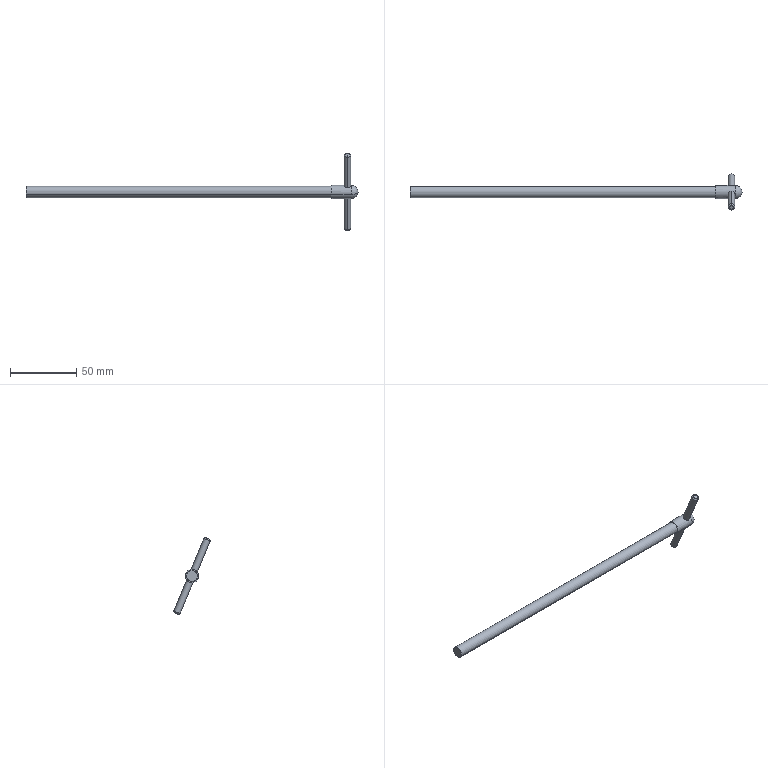Component | SolidWorks | TelescopicRod-1 | 2 solids | 20 faces | volume 15492 mm3 | cylinder 8 | torus 4 | plane 4 | cone 2 | sphere 2 | commonest cylinder face diameters 5 x4 8.5 x2 10 x2
build123d program:
from build123d import *

# Parameters (mm, degrees)
SKETCH1_R           = 5
BOSS_EXTRUDE1_DEPTH = 250
FILLET1_R           = 5
SKETCH2_R           = 2.5
CUT_EXTRUDE1_DEPTH  = 125
SKETCH3_R           = 2.5
BOSS_EXTRUDE2_DEPTH = 30.5
FILLET2_R           = 1
CHAMFER1_SIZE       = 1
SKETCH4_R           = 5.944
SKETCH4_R_2         = 4.25
CUT_EXTRUDE2_DEPTH  = 230


with BuildPart() as part:
    # Sketch1 → Boss-Extrude1 (new body)
    with BuildSketch(Plane(origin=(0, 0, 0), x_dir=(1, 0, 0), z_dir=(0, 1, 0))):
        with Locations(Location((0, 0, 0), (0, 0, 270))):
            Circle(SKETCH1_R)
    extrude(amount=BOSS_EXTRUDE1_DEPTH)

    # Fillet1
    fillet1_edges = [part.edges().sort_by_distance(p)[0] for p in [
        (0, 0, -5),
    ]]
    fillet(fillet1_edges, radius=FILLET1_R)

    # Sketch2 → Cut-Extrude1 (cut, symmetric)
    with BuildSketch(Plane(origin=(0, 0, 0), x_dir=(0, 0, -1), z_dir=(1, 0, 0))):
        with Locations((0, 8)):
            Circle(SKETCH2_R)
    extrude(amount=CUT_EXTRUDE1_DEPTH, both=True, mode=Mode.SUBTRACT)

    # Chamfer1
    chamfer1_edges = [part.edges().sort_by_distance(p)[0] for p in [
        (0, 250, -5),
    ]]
    chamfer(chamfer1_edges, length=CHAMFER1_SIZE)

    # Sketch4 → Cut-Extrude2 (cut)
    with BuildSketch(Plane(origin=(0, 250, 0), x_dir=(1, 0, 0), z_dir=(0, 1, 0))):
        Circle(SKETCH4_R)
        with Locations(Location((0, 0, 0), (0, 0, 270))):
            Circle(SKETCH4_R_2, mode=Mode.SUBTRACT)
    extrude(amount=-CUT_EXTRUDE2_DEPTH, mode=Mode.SUBTRACT)


with BuildPart() as body_2:
    # Sketch3 → Boss-Extrude2 (new, symmetric)
    with BuildSketch(Plane(origin=(0, 0, 0), x_dir=(0, 0, -1), z_dir=(1, 0, 0))):
        with Locations(Location((0, 8, 0), (0, 0, 180))):
            Circle(SKETCH3_R)
    extrude(amount=BOSS_EXTRUDE2_DEPTH, both=True)

    # Fillet2
    fillet2_edges = [body_2.edges().sort_by_distance(p)[0] for p in [
        (-30.5, 8, -2.5),
        (30.5, 8, -2.5),
    ]]
    fillet(fillet2_edges, radius=FILLET2_R)


solid = Compound([part.part, body_2.part])

# Placed as in the assembly
solid = solid.moved(Location((329.124, 2.944, 18.763), (112.448, 0, 90)))
STEP:
#1=COLOUR_RGB('',0.7922,0.8196,0.9333);
#2=FILL_AREA_STYLE_COLOUR('',#1);
#3=FILL_AREA_STYLE('',(#2));
#4=SURFACE_STYLE_FILL_AREA(#3);
#5=SURFACE_SIDE_STYLE('',(#4));
#6=SURFACE_STYLE_USAGE(.BOTH.,#5);
#7=PRESENTATION_STYLE_ASSIGNMENT((#6));
#8=CARTESIAN_POINT('',(3.115,-0.02963,0.6786));
#9=VERTEX_POINT('',#8);
#10=CARTESIAN_POINT('',(3.115,0.2615,0.7988));
#11=VERTEX_POINT('',#10);
#12=CARTESIAN_POINT('',(3.115,0.1159,0.7387));
#13=DIRECTION('',(-1.,0.,0.));
#14=DIRECTION('',(0.,-0.9242,-0.3818));
#15=AXIS2_PLACEMENT_3D('',#12,#13,#14);
#16=CIRCLE('',#15,0.1575);
#17=EDGE_CURVE('',#9,#11,#16,.T.);
#18=ORIENTED_EDGE('',*,*,#17,.F.);
#19=CARTESIAN_POINT('',(3.125,-0.03873,0.6748));
#20=VERTEX_POINT('',#19);
#21=CARTESIAN_POINT('',(3.115,-0.02963,0.6786));
#22=DIRECTION('',(0.7071,-0.6535,-0.27));
#23=VECTOR('',#22,39.37);
#24=LINE('',#21,#23);
#25=EDGE_CURVE('',#9,#20,#24,.T.);
#26=ORIENTED_EDGE('',*,*,#25,.T.);
#27=CARTESIAN_POINT('',(3.125,0.2706,0.8026));
#28=VERTEX_POINT('',#27);
#29=CARTESIAN_POINT('',(3.125,0.1159,0.7387));
#30=DIRECTION('',(-1.,0.,0.));
#31=DIRECTION('',(0.,0.9242,0.3818));
#32=AXIS2_PLACEMENT_3D('',#29,#30,#31);
#33=CIRCLE('',#32,0.1673);
#34=EDGE_CURVE('',#20,#28,#33,.T.);
#35=ORIENTED_EDGE('',*,*,#34,.T.);
#36=CARTESIAN_POINT('',(3.115,0.2615,0.7988));
#37=DIRECTION('',(0.7071,0.6535,0.27));
#38=VECTOR('',#37,39.37);
#39=LINE('',#36,#38);
#40=EDGE_CURVE('',#11,#28,#39,.T.);
#41=ORIENTED_EDGE('',*,*,#40,.F.);
#42=EDGE_LOOP('',(#18,#26,#35,#41));
#43=FACE_OUTER_BOUND('',#42,.T.);
#44=CARTESIAN_POINT('',(3.115,0.1159,0.7387));
#45=DIRECTION('',(1.,0.,0.));
#46=DIRECTION('',(0.,0.9242,0.3818));
#47=AXIS2_PLACEMENT_3D('',#44,#45,#46);
#48=CONICAL_SURFACE('',#47,0.1575,0.7854);
#49=ADVANCED_FACE('',(#43),#48,.T.);
#50=CARTESIAN_POINT('',(12.17,-0.03873,0.6748));
#51=VERTEX_POINT('',#50);
#52=CARTESIAN_POINT('',(12.17,0.2706,0.8026));
#53=VERTEX_POINT('',#52);
#54=CARTESIAN_POINT('',(12.17,0.1159,0.7387));
#55=DIRECTION('',(-1.,0.,0.));
#56=DIRECTION('',(0.,-0.9242,-0.3818));
#57=AXIS2_PLACEMENT_3D('',#54,#55,#56);
#58=CIRCLE('',#57,0.1673);
#59=EDGE_CURVE('',#51,#53,#58,.T.);
#60=ORIENTED_EDGE('',*,*,#59,.T.);
#61=CARTESIAN_POINT('',(12.17,0.2706,0.8026));
#62=DIRECTION('',(-1.,0.,0.));
#63=VECTOR('',#62,39.37);
#64=LINE('',#61,#63);
#65=EDGE_CURVE('',#53,#28,#64,.T.);
#66=ORIENTED_EDGE('',*,*,#65,.T.);
#67=ORIENTED_EDGE('',*,*,#34,.F.);
#68=CARTESIAN_POINT('',(12.17,-0.03873,0.6748));
#69=DIRECTION('',(-1.,0.,0.));
#70=VECTOR('',#69,39.37);
#71=LINE('',#68,#70);
#72=EDGE_CURVE('',#51,#20,#71,.T.);
#73=ORIENTED_EDGE('',*,*,#72,.F.);
#74=EDGE_LOOP('',(#60,#66,#67,#73));
#75=FACE_OUTER_BOUND('',#74,.T.);
#76=CARTESIAN_POINT('',(12.17,0.1159,0.7387));
#77=DIRECTION('',(-1.,0.,0.));
#78=DIRECTION('',(0.,-0.9242,-0.3818));
#79=AXIS2_PLACEMENT_3D('',#76,#77,#78);
#80=CYLINDRICAL_SURFACE('',#79,0.1673);
#81=ADVANCED_FACE('',(#75),#80,.T.);
#82=CARTESIAN_POINT('',(12.643,0.09005,0.5435));
#83=VERTEX_POINT('',#82);
#84=CARTESIAN_POINT('',(12.643,0.272,0.6187));
#85=VERTEX_POINT('',#84);
#86=CARTESIAN_POINT('',(12.643,0.09005,0.5435));
#87=CARTESIAN_POINT('',(12.649,0.09005,0.5435));
#88=CARTESIAN_POINT('',(12.656,0.09081,0.5434));
#89=CARTESIAN_POINT('',(12.669,0.09375,0.5431));
#90=CARTESIAN_POINT('',(12.675,0.09591,0.5428));
#91=CARTESIAN_POINT('',(12.687,0.1015,0.5423));
#92=CARTESIAN_POINT('',(12.692,0.1049,0.5421));
#93=CARTESIAN_POINT('',(12.703,0.1127,0.5418));
#94=CARTESIAN_POINT('',(12.708,0.1171,0.5418));
#95=CARTESIAN_POINT('',(12.717,0.1267,0.5421));
#96=CARTESIAN_POINT('',(12.721,0.1318,0.5424));
#97=CARTESIAN_POINT('',(12.728,0.1428,0.5436));
#98=CARTESIAN_POINT('',(12.731,0.1486,0.5445));
#99=CARTESIAN_POINT('',(12.736,0.1604,0.5468));
#100=CARTESIAN_POINT('',(12.738,0.1664,0.5483));
#101=CARTESIAN_POINT('',(12.74,0.1788,0.552));
#102=CARTESIAN_POINT('',(12.741,0.185,0.5542));
#103=CARTESIAN_POINT('',(12.741,0.197,0.5592));
#104=CARTESIAN_POINT('',(12.74,0.203,0.562));
#105=CARTESIAN_POINT('',(12.738,0.2144,0.5681));
#106=CARTESIAN_POINT('',(12.736,0.2197,0.5713));
#107=CARTESIAN_POINT('',(12.728,0.2349,0.5814));
#108=CARTESIAN_POINT('',(12.721,0.2436,0.5885));
#109=CARTESIAN_POINT('',(12.708,0.2541,0.5984));
#110=CARTESIAN_POINT('',(12.703,0.2571,0.6015));
#111=CARTESIAN_POINT('',(12.692,0.2624,0.6072));
#112=CARTESIAN_POINT('',(12.687,0.2647,0.6098));
#113=CARTESIAN_POINT('',(12.675,0.2683,0.614));
#114=CARTESIAN_POINT('',(12.669,0.2697,0.6157));
#115=CARTESIAN_POINT('',(12.656,0.2715,0.6181));
#116=CARTESIAN_POINT('',(12.649,0.272,0.6187));
#117=CARTESIAN_POINT('',(12.643,0.272,0.6187));
#118=B_SPLINE_CURVE_WITH_KNOTS('',3,(#86,#87,#88,#89,#90,#91,#92,#93,#94,#95,#96,#97,#98,#99,#100,#101,#102,#103,#104,#105,#106,#107,#108,#109,#110,#111,#112,#113,#114,#115,#116,#117),.UNSPECIFIED.,.F.,.F.,(4,2,2,2,2,2,2,2,2,2,2,2,2,2,2,4),(0.007951,0.008448,0.008944,0.00944,0.009936,0.01043,0.01093,0.01142,0.01192,0.01242,0.01291,0.0139,0.0144,0.0149,0.01539,0.01589),.UNSPECIFIED.);
#119=EDGE_CURVE('',#83,#85,#118,.T.);
#120=ORIENTED_EDGE('',*,*,#119,.F.);
#121=CARTESIAN_POINT('',(12.643,-0.04014,0.8587));
#122=VERTEX_POINT('',#121);
#123=CARTESIAN_POINT('',(12.643,1.904,-3.847));
#124=DIRECTION('',(0.,-0.3818,0.9242));
#125=VECTOR('',#124,39.37);
#126=LINE('',#123,#125);
#127=EDGE_CURVE('',#83,#122,#126,.T.);
#128=ORIENTED_EDGE('',*,*,#127,.T.);
#129=CARTESIAN_POINT('',(12.643,0.1418,0.9338));
#130=VERTEX_POINT('',#129);
#131=CARTESIAN_POINT('',(12.643,0.1418,0.9338));
#132=CARTESIAN_POINT('',(12.649,0.1418,0.9338));
#133=CARTESIAN_POINT('',(12.656,0.141,0.9339));
#134=CARTESIAN_POINT('',(12.669,0.1381,0.9343));
#135=CARTESIAN_POINT('',(12.675,0.1359,0.9345));
#136=CARTESIAN_POINT('',(12.693,0.1275,0.9353));
#137=CARTESIAN_POINT('',(12.703,0.1195,0.9357));
#138=CARTESIAN_POINT('',(12.717,0.1052,0.9353));
#139=CARTESIAN_POINT('',(12.721,0.09999,0.935));
#140=CARTESIAN_POINT('',(12.728,0.089,0.9338));
#141=CARTESIAN_POINT('',(12.731,0.08329,0.9329));
#142=CARTESIAN_POINT('',(12.736,0.07147,0.9305));
#143=CARTESIAN_POINT('',(12.738,0.06527,0.929));
#144=CARTESIAN_POINT('',(12.74,0.05298,0.9253));
#145=CARTESIAN_POINT('',(12.741,0.04687,0.9231));
#146=CARTESIAN_POINT('',(12.741,0.03475,0.9181));
#147=CARTESIAN_POINT('',(12.74,0.02875,0.9153));
#148=CARTESIAN_POINT('',(12.738,0.01745,0.9093));
#149=CARTESIAN_POINT('',(12.736,0.01202,0.906));
#150=CARTESIAN_POINT('',(12.731,0.001877,0.8993));
#151=CARTESIAN_POINT('',(12.728,-0.002784,0.8958));
#152=CARTESIAN_POINT('',(12.721,-0.01139,0.8889));
#153=CARTESIAN_POINT('',(12.717,-0.01533,0.8855));
#154=CARTESIAN_POINT('',(12.703,-0.02576,0.8757));
#155=CARTESIAN_POINT('',(12.692,-0.03112,0.8697));
#156=CARTESIAN_POINT('',(12.675,-0.03648,0.8633));
#157=CARTESIAN_POINT('',(12.669,-0.03786,0.8616));
#158=CARTESIAN_POINT('',(12.656,-0.03969,0.8593));
#159=CARTESIAN_POINT('',(12.649,-0.04014,0.8587));
#160=CARTESIAN_POINT('',(12.643,-0.04014,0.8587));
#161=B_SPLINE_CURVE_WITH_KNOTS('',3,(#131,#132,#133,#134,#135,#136,#137,#138,#139,#140,#141,#142,#143,#144,#145,#146,#147,#148,#149,#150,#151,#152,#153,#154,#155,#156,#157,#158,#159,#160),.UNSPECIFIED.,.F.,.F.,(4,2,2,2,2,2,2,2,2,2,2,2,2,2,4),(0.,0.000497,0.0009939,0.001988,0.002485,0.002982,0.003479,0.003976,0.004473,0.00497,0.005467,0.005964,0.006958,0.007455,0.007951),.UNSPECIFIED.);
#162=EDGE_CURVE('',#130,#122,#161,.T.);
#163=ORIENTED_EDGE('',*,*,#162,.F.);
#164=CARTESIAN_POINT('',(12.643,2.086,-3.772));
#165=DIRECTION('',(0.,-0.3818,0.9242));
#166=VECTOR('',#165,39.37);
#167=LINE('',#164,#166);
#168=EDGE_CURVE('',#85,#130,#167,.T.);
#169=ORIENTED_EDGE('',*,*,#168,.F.);
#170=EDGE_LOOP('',(#120,#128,#163,#169));
#171=FACE_OUTER_BOUND('',#170,.T.);
#172=CARTESIAN_POINT('',(12.643,1.995,-3.81));
#173=DIRECTION('',(0.,-0.3818,0.9242));
#174=DIRECTION('',(0.,0.9242,0.3818));
#175=AXIS2_PLACEMENT_3D('',#172,#173,#174);
#176=CYLINDRICAL_SURFACE('',#175,0.09843);
#177=ADVANCED_FACE('',(#171),#176,.F.);
#178=CARTESIAN_POINT('',(12.958,0.1159,0.7387));
#179=VERTEX_POINT('',#178);
#180=CARTESIAN_POINT('',(12.761,-0.06602,0.6635));
#181=VERTEX_POINT('',#180);
#182=CARTESIAN_POINT('',(12.761,0.1159,0.7387));
#183=DIRECTION('',(0.,0.3818,-0.9242));
#184=DIRECTION('',(0.,0.9242,0.3818));
#185=AXIS2_PLACEMENT_3D('',#182,#183,#184);
#186=CIRCLE('',#185,0.1969);
#187=EDGE_CURVE('',#179,#181,#186,.T.);
#188=ORIENTED_EDGE('',*,*,#187,.F.);
#189=CARTESIAN_POINT('',(12.761,0.2979,0.8139));
#190=VERTEX_POINT('',#189);
#191=CARTESIAN_POINT('',(12.761,0.1159,0.7387));
#192=DIRECTION('',(0.,-0.3818,0.9242));
#193=DIRECTION('',(0.,-0.9242,-0.3818));
#194=AXIS2_PLACEMENT_3D('',#191,#192,#193);
#195=CIRCLE('',#194,0.1969);
#196=EDGE_CURVE('',#179,#190,#195,.T.);
#197=ORIENTED_EDGE('',*,*,#196,.T.);
#198=CARTESIAN_POINT('',(12.761,0.1159,0.7387));
#199=DIRECTION('',(-1.,0.,0.));
#200=DIRECTION('',(0.,0.9242,0.3818));
#201=AXIS2_PLACEMENT_3D('',#198,#199,#200);
#202=CIRCLE('',#201,0.1969);
#203=EDGE_CURVE('',#181,#190,#202,.T.);
#204=ORIENTED_EDGE('',*,*,#203,.F.);
#205=EDGE_LOOP('',(#188,#197,#204));
#206=FACE_OUTER_BOUND('',#205,.T.);
#207=CARTESIAN_POINT('',(12.761,0.1159,0.7387));
#208=DIRECTION('',(0.,-0.3818,0.9242));
#209=DIRECTION('',(0.,-0.9242,-0.3818));
#210=AXIS2_PLACEMENT_3D('',#207,#208,#209);
#211=SPHERICAL_SURFACE('',#210,0.1969);
#212=ADVANCED_FACE('',(#206),#211,.T.);
#213=ORIENTED_EDGE('',*,*,#162,.T.);
#214=CARTESIAN_POINT('',(12.643,-0.04014,0.8587));
#215=CARTESIAN_POINT('',(12.636,-0.04014,0.8587));
#216=CARTESIAN_POINT('',(12.63,-0.03968,0.8593));
#217=CARTESIAN_POINT('',(12.617,-0.03785,0.8616));
#218=CARTESIAN_POINT('',(12.611,-0.03649,0.8633));
#219=CARTESIAN_POINT('',(12.599,-0.03286,0.8676));
#220=CARTESIAN_POINT('',(12.593,-0.03063,0.8702));
#221=CARTESIAN_POINT('',(12.583,-0.02532,0.8759));
#222=CARTESIAN_POINT('',(12.578,-0.02221,0.879));
#223=CARTESIAN_POINT('',(12.569,-0.01524,0.8856));
#224=CARTESIAN_POINT('',(12.565,-0.01137,0.8889));
#225=CARTESIAN_POINT('',(12.557,-0.002769,0.8958));
#226=CARTESIAN_POINT('',(12.554,0.001971,0.8993));
#227=CARTESIAN_POINT('',(12.549,0.012,0.906));
#228=CARTESIAN_POINT('',(12.548,0.01733,0.9092));
#229=CARTESIAN_POINT('',(12.545,0.02873,0.9153));
#230=CARTESIAN_POINT('',(12.544,0.03465,0.9181));
#231=CARTESIAN_POINT('',(12.544,0.04669,0.9231));
#232=CARTESIAN_POINT('',(12.545,0.05293,0.9253));
#233=CARTESIAN_POINT('',(12.547,0.06526,0.929));
#234=CARTESIAN_POINT('',(12.549,0.07133,0.9305));
#235=CARTESIAN_POINT('',(12.557,0.08922,0.9341));
#236=CARTESIAN_POINT('',(12.564,0.1004,0.9352));
#237=CARTESIAN_POINT('',(12.578,0.1148,0.9356));
#238=CARTESIAN_POINT('',(12.583,0.1191,0.9356));
#239=CARTESIAN_POINT('',(12.593,0.1269,0.9353));
#240=CARTESIAN_POINT('',(12.599,0.1303,0.935));
#241=CARTESIAN_POINT('',(12.611,0.1359,0.9345));
#242=CARTESIAN_POINT('',(12.617,0.1381,0.9343));
#243=CARTESIAN_POINT('',(12.629,0.141,0.9339));
#244=CARTESIAN_POINT('',(12.636,0.1418,0.9338));
#245=CARTESIAN_POINT('',(12.643,0.1418,0.9338));
#246=B_SPLINE_CURVE_WITH_KNOTS('',3,(#214,#215,#216,#217,#218,#219,#220,#221,#222,#223,#224,#225,#226,#227,#228,#229,#230,#231,#232,#233,#234,#235,#236,#237,#238,#239,#240,#241,#242,#243,#244,#245),.UNSPECIFIED.,.F.,.F.,(4,2,2,2,2,2,2,2,2,2,2,2,2,2,2,4),(0.007951,0.008448,0.008944,0.00944,0.009936,0.01043,0.01093,0.01142,0.01192,0.01242,0.01291,0.0139,0.0144,0.0149,0.01539,0.01589),.UNSPECIFIED.);
#247=EDGE_CURVE('',#122,#130,#246,.T.);
#248=ORIENTED_EDGE('',*,*,#247,.T.);
#249=EDGE_LOOP('',(#213,#248));
#250=FACE_BOUND('',#249,.T.);
#251=CARTESIAN_POINT('',(12.17,-0.06602,0.6635));
#252=VERTEX_POINT('',#251);
#253=CARTESIAN_POINT('',(12.17,0.2979,0.8139));
#254=VERTEX_POINT('',#253);
#255=CARTESIAN_POINT('',(12.17,0.1159,0.7387));
#256=DIRECTION('',(-1.,0.,0.));
#257=DIRECTION('',(0.,-0.9242,-0.3818));
#258=AXIS2_PLACEMENT_3D('',#255,#256,#257);
#259=CIRCLE('',#258,0.1969);
#260=EDGE_CURVE('',#252,#254,#259,.T.);
#261=ORIENTED_EDGE('',*,*,#260,.F.);
#262=CARTESIAN_POINT('',(3.115,-0.06602,0.6635));
#263=DIRECTION('',(1.,0.,0.));
#264=VECTOR('',#263,39.37);
#265=LINE('',#262,#264);
#266=EDGE_CURVE('',#252,#181,#265,.T.);
#267=ORIENTED_EDGE('',*,*,#266,.T.);
#268=ORIENTED_EDGE('',*,*,#203,.T.);
#269=CARTESIAN_POINT('',(3.115,0.2979,0.8139));
#270=DIRECTION('',(1.,0.,0.));
#271=VECTOR('',#270,39.37);
#272=LINE('',#269,#271);
#273=EDGE_CURVE('',#254,#190,#272,.T.);
#274=ORIENTED_EDGE('',*,*,#273,.F.);
#275=EDGE_LOOP('',(#261,#267,#268,#274));
#276=FACE_OUTER_BOUND('',#275,.T.);
#277=CARTESIAN_POINT('',(3.115,0.1159,0.7387));
#278=DIRECTION('',(1.,0.,0.));
#279=DIRECTION('',(0.,0.9242,0.3818));
#280=AXIS2_PLACEMENT_3D('',#277,#278,#279);
#281=CYLINDRICAL_SURFACE('',#280,0.1969);
#282=ADVANCED_FACE('',(#250,#276),#281,.T.);
#283=ORIENTED_EDGE('',*,*,#266,.F.);
#284=CARTESIAN_POINT('',(12.17,0.1159,0.7387));
#285=DIRECTION('',(-1.,0.,0.));
#286=DIRECTION('',(0.,-0.9242,-0.3818));
#287=AXIS2_PLACEMENT_3D('',#284,#285,#286);
#288=CIRCLE('',#287,0.1969);
#289=EDGE_CURVE('',#254,#252,#288,.T.);
#290=ORIENTED_EDGE('',*,*,#289,.F.);
#291=ORIENTED_EDGE('',*,*,#273,.T.);
#292=CARTESIAN_POINT('',(12.761,0.1159,0.7387));
#293=DIRECTION('',(-1.,0.,0.));
#294=DIRECTION('',(0.,0.9242,0.3818));
#295=AXIS2_PLACEMENT_3D('',#292,#293,#294);
#296=CIRCLE('',#295,0.1969);
#297=EDGE_CURVE('',#190,#181,#296,.T.);
#298=ORIENTED_EDGE('',*,*,#297,.T.);
#299=EDGE_LOOP('',(#283,#290,#291,#298));
#300=FACE_OUTER_BOUND('',#299,.T.);
#301=CARTESIAN_POINT('',(12.643,0.272,0.6187));
#302=CARTESIAN_POINT('',(12.636,0.272,0.6187));
#303=CARTESIAN_POINT('',(12.63,0.2715,0.6181));
#304=CARTESIAN_POINT('',(12.617,0.2697,0.6158));
#305=CARTESIAN_POINT('',(12.611,0.2683,0.6141));
#306=CARTESIAN_POINT('',(12.593,0.2629,0.6076));
#307=CARTESIAN_POINT('',(12.582,0.2575,0.6016));
#308=CARTESIAN_POINT('',(12.569,0.2471,0.5918));
#309=CARTESIAN_POINT('',(12.565,0.2432,0.5884));
#310=CARTESIAN_POINT('',(12.557,0.2345,0.5815));
#311=CARTESIAN_POINT('',(12.554,0.2299,0.5781));
#312=CARTESIAN_POINT('',(12.549,0.2199,0.5714));
#313=CARTESIAN_POINT('',(12.547,0.2144,0.5681));
#314=CARTESIAN_POINT('',(12.545,0.2031,0.5621));
#315=CARTESIAN_POINT('',(12.544,0.1972,0.5593));
#316=CARTESIAN_POINT('',(12.544,0.1851,0.5543));
#317=CARTESIAN_POINT('',(12.545,0.1788,0.5521));
#318=CARTESIAN_POINT('',(12.547,0.1666,0.5484));
#319=CARTESIAN_POINT('',(12.549,0.1604,0.5468));
#320=CARTESIAN_POINT('',(12.554,0.1485,0.5445));
#321=CARTESIAN_POINT('',(12.557,0.1427,0.5436));
#322=CARTESIAN_POINT('',(12.565,0.1318,0.5424));
#323=CARTESIAN_POINT('',(12.569,0.1266,0.5421));
#324=CARTESIAN_POINT('',(12.582,0.1123,0.5416));
#325=CARTESIAN_POINT('',(12.593,0.1042,0.5421));
#326=CARTESIAN_POINT('',(12.611,0.09592,0.5428));
#327=CARTESIAN_POINT('',(12.617,0.09373,0.5431));
#328=CARTESIAN_POINT('',(12.63,0.09079,0.5434));
#329=CARTESIAN_POINT('',(12.636,0.09005,0.5435));
#330=CARTESIAN_POINT('',(12.643,0.09005,0.5435));
#331=B_SPLINE_CURVE_WITH_KNOTS('',3,(#301,#302,#303,#304,#305,#306,#307,#308,#309,#310,#311,#312,#313,#314,#315,#316,#317,#318,#319,#320,#321,#322,#323,#324,#325,#326,#327,#328,#329,#330),.UNSPECIFIED.,.F.,.F.,(4,2,2,2,2,2,2,2,2,2,2,2,2,2,4),(0.,0.000497,0.0009939,0.001988,0.002485,0.002982,0.003479,0.003976,0.004473,0.00497,0.005467,0.005964,0.006958,0.007455,0.007951),.UNSPECIFIED.);
#332=EDGE_CURVE('',#85,#83,#331,.T.);
#333=ORIENTED_EDGE('',*,*,#332,.T.);
#334=ORIENTED_EDGE('',*,*,#119,.T.);
#335=EDGE_LOOP('',(#333,#334));
#336=FACE_BOUND('',#335,.T.);
#337=CARTESIAN_POINT('',(3.115,0.1159,0.7387));
#338=DIRECTION('',(1.,0.,0.));
#339=DIRECTION('',(0.,0.9242,0.3818));
#340=AXIS2_PLACEMENT_3D('',#337,#338,#339);
#341=CYLINDRICAL_SURFACE('',#340,0.1969);
#342=ADVANCED_FACE('',(#300,#336),#341,.T.);
#343=ORIENTED_EDGE('',*,*,#196,.F.);
#344=ORIENTED_EDGE('',*,*,#187,.T.);
#345=ORIENTED_EDGE('',*,*,#297,.F.);
#346=EDGE_LOOP('',(#343,#344,#345));
#347=FACE_OUTER_BOUND('',#346,.T.);
#348=CARTESIAN_POINT('',(12.761,0.1159,0.7387));
#349=DIRECTION('',(0.,-0.3818,0.9242));
#350=DIRECTION('',(0.,-0.9242,-0.3818));
#351=AXIS2_PLACEMENT_3D('',#348,#349,#350);
#352=SPHERICAL_SURFACE('',#351,0.1969);
#353=ADVANCED_FACE('',(#347),#352,.T.);
#354=ORIENTED_EDGE('',*,*,#127,.F.);
#355=ORIENTED_EDGE('',*,*,#332,.F.);
#356=ORIENTED_EDGE('',*,*,#168,.T.);
#357=ORIENTED_EDGE('',*,*,#247,.F.);
#358=EDGE_LOOP('',(#354,#355,#356,#357));
#359=FACE_OUTER_BOUND('',#358,.T.);
#360=CARTESIAN_POINT('',(12.643,1.995,-3.81));
#361=DIRECTION('',(0.,-0.3818,0.9242));
#362=DIRECTION('',(0.,0.9242,0.3818));
#363=AXIS2_PLACEMENT_3D('',#360,#361,#362);
#364=CYLINDRICAL_SURFACE('',#363,0.09843);
#365=ADVANCED_FACE('',(#359),#364,.F.);
#366=ORIENTED_EDGE('',*,*,#59,.F.);
#367=CARTESIAN_POINT('',(12.17,0.1159,0.7387));
#368=DIRECTION('',(-1.,0.,0.));
#369=DIRECTION('',(0.,-0.9242,-0.3818));
#370=AXIS2_PLACEMENT_3D('',#367,#368,#369);
#371=CIRCLE('',#370,0.1673);
#372=EDGE_CURVE('',#53,#51,#371,.T.);
#373=ORIENTED_EDGE('',*,*,#372,.F.);
#374=EDGE_LOOP('',(#366,#373));
#375=FACE_BOUND('',#374,.T.);
#376=ORIENTED_EDGE('',*,*,#289,.T.);
#377=ORIENTED_EDGE('',*,*,#260,.T.);
#378=EDGE_LOOP('',(#376,#377));
#379=FACE_OUTER_BOUND('',#378,.T.);
#380=CARTESIAN_POINT('',(12.17,0.1159,0.7387));
#381=DIRECTION('',(-1.,0.,0.));
#382=DIRECTION('',(0.,-0.9242,-0.3818));
#383=AXIS2_PLACEMENT_3D('',#380,#381,#382);
#384=PLANE('',#383);
#385=ADVANCED_FACE('',(#375,#379),#384,.T.);
#386=ORIENTED_EDGE('',*,*,#65,.F.);
#387=ORIENTED_EDGE('',*,*,#372,.T.);
#388=ORIENTED_EDGE('',*,*,#72,.T.);
#389=CARTESIAN_POINT('',(3.125,0.1159,0.7387));
#390=DIRECTION('',(-1.,0.,0.));
#391=DIRECTION('',(0.,0.9242,0.3818));
#392=AXIS2_PLACEMENT_3D('',#389,#390,#391);
#393=CIRCLE('',#392,0.1673);
#394=EDGE_CURVE('',#28,#20,#393,.T.);
#395=ORIENTED_EDGE('',*,*,#394,.F.);
#396=EDGE_LOOP('',(#386,#387,#388,#395));
#397=FACE_OUTER_BOUND('',#396,.T.);
#398=CARTESIAN_POINT('',(12.17,0.1159,0.7387));
#399=DIRECTION('',(-1.,0.,0.));
#400=DIRECTION('',(0.,-0.9242,-0.3818));
#401=AXIS2_PLACEMENT_3D('',#398,#399,#400);
#402=CYLINDRICAL_SURFACE('',#401,0.1673);
#403=ADVANCED_FACE('',(#397),#402,.T.);
#404=CARTESIAN_POINT('',(3.115,0.1159,0.7387));
#405=DIRECTION('',(-1.,0.,0.));
#406=DIRECTION('',(0.,-0.9242,-0.3818));
#407=AXIS2_PLACEMENT_3D('',#404,#405,#406);
#408=CIRCLE('',#407,0.1575);
#409=EDGE_CURVE('',#11,#9,#408,.T.);
#410=ORIENTED_EDGE('',*,*,#409,.T.);
#411=ORIENTED_EDGE('',*,*,#17,.T.);
#412=EDGE_LOOP('',(#410,#411));
#413=FACE_OUTER_BOUND('',#412,.T.);
#414=CARTESIAN_POINT('',(3.115,0.1159,0.7387));
#415=DIRECTION('',(-1.,0.,0.));
#416=DIRECTION('',(0.,-0.9242,-0.3818));
#417=AXIS2_PLACEMENT_3D('',#414,#415,#416);
#418=PLANE('',#417);
#419=ADVANCED_FACE('',(#413),#418,.T.);
#420=ORIENTED_EDGE('',*,*,#25,.F.);
#421=ORIENTED_EDGE('',*,*,#409,.F.);
#422=ORIENTED_EDGE('',*,*,#40,.T.);
#423=ORIENTED_EDGE('',*,*,#394,.T.);
#424=EDGE_LOOP('',(#420,#421,#422,#423));
#425=FACE_OUTER_BOUND('',#424,.T.);
#426=CARTESIAN_POINT('',(3.115,0.1159,0.7387));
#427=DIRECTION('',(1.,0.,0.));
#428=DIRECTION('',(0.,0.9242,0.3818));
#429=AXIS2_PLACEMENT_3D('',#426,#427,#428);
#430=CONICAL_SURFACE('',#429,0.1575,0.7854);
#431=ADVANCED_FACE('',(#425),#430,.T.);
#432=CLOSED_SHELL('',(#49,#81,#177,#212,#282,#342,#353,#365,#385,#403,#419,#431));
#433=MANIFOLD_SOLID_BREP('',#432);
#434=STYLED_ITEM('',(#7),#433);
#435=(LENGTH_UNIT()NAMED_UNIT(*)SI_UNIT($,.METRE.));
#436=LENGTH_MEASURE_WITH_UNIT(LENGTH_MEASURE(0.0254),#435);
#437=DIMENSIONAL_EXPONENTS(1.,0.,0.,0.,0.,0.,0.);
#438=(CONVERSION_BASED_UNIT('',#436)LENGTH_UNIT()NAMED_UNIT(#437));
#439=UNCERTAINTY_MEASURE_WITH_UNIT(LENGTH_MEASURE(0.00001),#438,'','');
#440=(NAMED_UNIT(*)PLANE_ANGLE_UNIT()SI_UNIT($,.RADIAN.));
#441=(NAMED_UNIT(*)SI_UNIT($,.STERADIAN.)SOLID_ANGLE_UNIT());
#442=(GEOMETRIC_REPRESENTATION_CONTEXT(3)GLOBAL_UNCERTAINTY_ASSIGNED_CONTEXT((#439))GLOBAL_UNIT_ASSIGNED_CONTEXT((#438,#440,#441))REPRESENTATION_CONTEXT('',''));
#443=MECHANICAL_DESIGN_GEOMETRIC_PRESENTATION_REPRESENTATION('',(#434),#442);
#444=PRESENTATION_LAYER_ASSIGNMENT('','',(#434));
#445=COLOUR_RGB('',0.7922,0.8196,0.9333);
#446=FILL_AREA_STYLE_COLOUR('',#445);
#447=FILL_AREA_STYLE('',(#446));
#448=SURFACE_STYLE_FILL_AREA(#447);
#449=SURFACE_SIDE_STYLE('',(#448));
#450=SURFACE_STYLE_USAGE(.BOTH.,#449);
#451=PRESENTATION_STYLE_ASSIGNMENT((#450));
#452=CARTESIAN_POINT('',(12.643,-0.4185,1.775));
#453=VERTEX_POINT('',#452);
#454=CARTESIAN_POINT('',(12.643,-0.2366,1.85));
#455=VERTEX_POINT('',#454);
#456=CARTESIAN_POINT('',(12.643,-0.3276,1.812));
#457=DIRECTION('',(0.,0.3818,-0.9242));
#458=DIRECTION('',(0.,0.9242,0.3818));
#459=AXIS2_PLACEMENT_3D('',#456,#457,#458);
#460=CIRCLE('',#459,0.09843);
#461=EDGE_CURVE('',#453,#455,#460,.T.);
#462=ORIENTED_EDGE('',*,*,#461,.F.);
#463=CARTESIAN_POINT('',(12.643,-0.3972,1.826));
#464=VERTEX_POINT('',#463);
#465=CARTESIAN_POINT('',(12.643,-0.3821,1.79));
#466=DIRECTION('',(-1.,0.,0.));
#467=DIRECTION('',(0.,-1.,0.));
#468=AXIS2_PLACEMENT_3D('',#465,#466,#467);
#469=CIRCLE('',#468,0.03937);
#470=EDGE_CURVE('',#453,#464,#469,.T.);
#471=ORIENTED_EDGE('',*,*,#470,.T.);
#472=CARTESIAN_POINT('',(12.643,-0.288,1.871));
#473=VERTEX_POINT('',#472);
#474=CARTESIAN_POINT('',(12.643,-0.3426,1.848));
#475=DIRECTION('',(0.,-0.3818,0.9242));
#476=DIRECTION('',(0.,0.9242,0.3818));
#477=AXIS2_PLACEMENT_3D('',#474,#475,#476);
#478=CIRCLE('',#477,0.05906);
#479=EDGE_CURVE('',#473,#464,#478,.T.);
#480=ORIENTED_EDGE('',*,*,#479,.F.);
#481=CARTESIAN_POINT('',(12.643,-0.273,1.835));
#482=DIRECTION('',(1.,0.,0.));
#483=DIRECTION('',(0.,0.,-1.));
#484=AXIS2_PLACEMENT_3D('',#481,#482,#483);
#485=CIRCLE('',#484,0.03937);
#486=EDGE_CURVE('',#455,#473,#485,.T.);
#487=ORIENTED_EDGE('',*,*,#486,.F.);
#488=EDGE_LOOP('',(#462,#471,#480,#487));
#489=FACE_OUTER_BOUND('',#488,.T.);
#490=CARTESIAN_POINT('',(12.643,-0.3276,1.812));
#491=DIRECTION('',(0.,-0.3818,0.9242));
#492=DIRECTION('',(0.,0.9242,0.3818));
#493=AXIS2_PLACEMENT_3D('',#490,#491,#492);
#494=TOROIDAL_SURFACE('',#493,0.05906,0.03937);
#495=ADVANCED_FACE('',(#489),#494,.T.);
#496=CARTESIAN_POINT('',(12.643,0.5199,-0.3937));
#497=VERTEX_POINT('',#496);
#498=CARTESIAN_POINT('',(12.643,0.629,-0.3486));
#499=VERTEX_POINT('',#498);
#500=CARTESIAN_POINT('',(12.643,0.5744,-0.3711));
#501=DIRECTION('',(0.,0.3818,-0.9242));
#502=DIRECTION('',(0.,0.9242,0.3818));
#503=AXIS2_PLACEMENT_3D('',#500,#501,#502);
#504=CIRCLE('',#503,0.05906);
#505=EDGE_CURVE('',#497,#499,#504,.T.);
#506=ORIENTED_EDGE('',*,*,#505,.F.);
#507=CARTESIAN_POINT('',(12.643,0.4684,-0.3723));
#508=VERTEX_POINT('',#507);
#509=CARTESIAN_POINT('',(12.643,0.5048,-0.3573));
#510=DIRECTION('',(-1.,0.,0.));
#511=DIRECTION('',(0.,-1.,0.));
#512=AXIS2_PLACEMENT_3D('',#509,#510,#511);
#513=CIRCLE('',#512,0.03937);
#514=EDGE_CURVE('',#497,#508,#513,.T.);
#515=ORIENTED_EDGE('',*,*,#514,.T.);
#516=CARTESIAN_POINT('',(12.643,0.6504,-0.2971));
#517=VERTEX_POINT('',#516);
#518=CARTESIAN_POINT('',(12.643,0.5594,-0.3347));
#519=DIRECTION('',(0.,-0.3818,0.9242));
#520=DIRECTION('',(0.,0.9242,0.3818));
#521=AXIS2_PLACEMENT_3D('',#518,#519,#520);
#522=CIRCLE('',#521,0.09843);
#523=EDGE_CURVE('',#517,#508,#522,.T.);
#524=ORIENTED_EDGE('',*,*,#523,.F.);
#525=CARTESIAN_POINT('',(12.643,0.614,-0.3122));
#526=DIRECTION('',(1.,0.,0.));
#527=DIRECTION('',(0.,0.,-1.));
#528=AXIS2_PLACEMENT_3D('',#525,#526,#527);
#529=CIRCLE('',#528,0.03937);
#530=EDGE_CURVE('',#499,#517,#529,.T.);
#531=ORIENTED_EDGE('',*,*,#530,.F.);
#532=EDGE_LOOP('',(#506,#515,#524,#531));
#533=FACE_OUTER_BOUND('',#532,.T.);
#534=CARTESIAN_POINT('',(12.643,0.5594,-0.3347));
#535=DIRECTION('',(0.,-0.3818,0.9242));
#536=DIRECTION('',(0.,0.9242,0.3818));
#537=AXIS2_PLACEMENT_3D('',#534,#535,#536);
#538=TOROIDAL_SURFACE('',#537,0.05906,0.03937);
#539=ADVANCED_FACE('',(#533),#538,.T.);
#540=ORIENTED_EDGE('',*,*,#461,.T.);
#541=CARTESIAN_POINT('',(12.643,-0.2516,1.886));
#542=DIRECTION('',(0.,0.3818,-0.9242));
#543=VECTOR('',#542,39.37);
#544=LINE('',#541,#543);
#545=EDGE_CURVE('',#455,#517,#544,.T.);
#546=ORIENTED_EDGE('',*,*,#545,.T.);
#547=ORIENTED_EDGE('',*,*,#523,.T.);
#548=CARTESIAN_POINT('',(12.643,-0.4336,1.811));
#549=DIRECTION('',(0.,0.3818,-0.9242));
#550=VECTOR('',#549,39.37);
#551=LINE('',#548,#550);
#552=EDGE_CURVE('',#453,#508,#551,.T.);
#553=ORIENTED_EDGE('',*,*,#552,.F.);
#554=EDGE_LOOP('',(#540,#546,#547,#553));
#555=FACE_OUTER_BOUND('',#554,.T.);
#556=CARTESIAN_POINT('',(12.643,-0.3426,1.848));
#557=DIRECTION('',(0.,0.3818,-0.9242));
#558=DIRECTION('',(0.,-0.9242,-0.3818));
#559=AXIS2_PLACEMENT_3D('',#556,#557,#558);
#560=CYLINDRICAL_SURFACE('',#559,0.09843);
#561=ADVANCED_FACE('',(#555),#560,.T.);
#562=ORIENTED_EDGE('',*,*,#545,.F.);
#563=CARTESIAN_POINT('',(12.643,-0.3276,1.812));
#564=DIRECTION('',(0.,0.3818,-0.9242));
#565=DIRECTION('',(0.,0.9242,0.3818));
#566=AXIS2_PLACEMENT_3D('',#563,#564,#565);
#567=CIRCLE('',#566,0.09843);
#568=EDGE_CURVE('',#455,#453,#567,.T.);
#569=ORIENTED_EDGE('',*,*,#568,.T.);
#570=ORIENTED_EDGE('',*,*,#552,.T.);
#571=CARTESIAN_POINT('',(12.643,0.5594,-0.3347));
#572=DIRECTION('',(0.,-0.3818,0.9242));
#573=DIRECTION('',(0.,0.9242,0.3818));
#574=AXIS2_PLACEMENT_3D('',#571,#572,#573);
#575=CIRCLE('',#574,0.09843);
#576=EDGE_CURVE('',#508,#517,#575,.T.);
#577=ORIENTED_EDGE('',*,*,#576,.T.);
#578=EDGE_LOOP('',(#562,#569,#570,#577));
#579=FACE_OUTER_BOUND('',#578,.T.);
#580=CARTESIAN_POINT('',(12.643,-0.3426,1.848));
#581=DIRECTION('',(0.,0.3818,-0.9242));
#582=DIRECTION('',(0.,-0.9242,-0.3818));
#583=AXIS2_PLACEMENT_3D('',#580,#581,#582);
#584=CYLINDRICAL_SURFACE('',#583,0.09843);
#585=ADVANCED_FACE('',(#579),#584,.T.);
#586=ORIENTED_EDGE('',*,*,#479,.T.);
#587=CARTESIAN_POINT('',(12.643,-0.3426,1.848));
#588=DIRECTION('',(0.,-0.3818,0.9242));
#589=DIRECTION('',(0.,0.9242,0.3818));
#590=AXIS2_PLACEMENT_3D('',#587,#588,#589);
#591=CIRCLE('',#590,0.05906);
#592=EDGE_CURVE('',#464,#473,#591,.T.);
#593=ORIENTED_EDGE('',*,*,#592,.T.);
#594=EDGE_LOOP('',(#586,#593));
#595=FACE_OUTER_BOUND('',#594,.T.);
#596=CARTESIAN_POINT('',(12.643,-0.3426,1.848));
#597=DIRECTION('',(0.,-0.3818,0.9242));
#598=DIRECTION('',(0.,0.9242,0.3818));
#599=AXIS2_PLACEMENT_3D('',#596,#597,#598);
#600=PLANE('',#599);
#601=ADVANCED_FACE('',(#595),#600,.T.);
#602=CARTESIAN_POINT('',(12.643,0.5744,-0.3711));
#603=DIRECTION('',(0.,0.3818,-0.9242));
#604=DIRECTION('',(0.,0.9242,0.3818));
#605=AXIS2_PLACEMENT_3D('',#602,#603,#604);
#606=CIRCLE('',#605,0.05906);
#607=EDGE_CURVE('',#499,#497,#606,.T.);
#608=ORIENTED_EDGE('',*,*,#607,.T.);
#609=ORIENTED_EDGE('',*,*,#505,.T.);
#610=EDGE_LOOP('',(#608,#609));
#611=FACE_OUTER_BOUND('',#610,.T.);
#612=CARTESIAN_POINT('',(12.643,0.5744,-0.3711));
#613=DIRECTION('',(0.,-0.3818,0.9242));
#614=DIRECTION('',(0.,0.9242,0.3818));
#615=AXIS2_PLACEMENT_3D('',#612,#613,#614);
#616=PLANE('',#615);
#617=ADVANCED_FACE('',(#611),#616,.F.);
#618=ORIENTED_EDGE('',*,*,#514,.F.);
#619=ORIENTED_EDGE('',*,*,#607,.F.);
#620=ORIENTED_EDGE('',*,*,#530,.T.);
#621=ORIENTED_EDGE('',*,*,#576,.F.);
#622=EDGE_LOOP('',(#618,#619,#620,#621));
#623=FACE_OUTER_BOUND('',#622,.T.);
#624=CARTESIAN_POINT('',(12.643,0.5594,-0.3347));
#625=DIRECTION('',(0.,-0.3818,0.9242));
#626=DIRECTION('',(0.,0.9242,0.3818));
#627=AXIS2_PLACEMENT_3D('',#624,#625,#626);
#628=TOROIDAL_SURFACE('',#627,0.05906,0.03937);
#629=ADVANCED_FACE('',(#623),#628,.T.);
#630=ORIENTED_EDGE('',*,*,#470,.F.);
#631=ORIENTED_EDGE('',*,*,#568,.F.);
#632=ORIENTED_EDGE('',*,*,#486,.T.);
#633=ORIENTED_EDGE('',*,*,#592,.F.);
#634=EDGE_LOOP('',(#630,#631,#632,#633));
#635=FACE_OUTER_BOUND('',#634,.T.);
#636=CARTESIAN_POINT('',(12.643,-0.3276,1.812));
#637=DIRECTION('',(0.,-0.3818,0.9242));
#638=DIRECTION('',(0.,0.9242,0.3818));
#639=AXIS2_PLACEMENT_3D('',#636,#637,#638);
#640=TOROIDAL_SURFACE('',#639,0.05906,0.03937);
#641=ADVANCED_FACE('',(#635),#640,.T.);
#642=CLOSED_SHELL('',(#495,#539,#561,#585,#601,#617,#629,#641));
#643=MANIFOLD_SOLID_BREP('',#642);
#644=STYLED_ITEM('',(#451),#643);
#645=PRESENTATION_LAYER_ASSIGNMENT('','',(#644));
#646=(LENGTH_UNIT()NAMED_UNIT(*)SI_UNIT($,.METRE.));
#647=LENGTH_MEASURE_WITH_UNIT(LENGTH_MEASURE(0.0254),#646);
#648=DIMENSIONAL_EXPONENTS(1.,0.,0.,0.,0.,0.,0.);
#649=(CONVERSION_BASED_UNIT('',#647)LENGTH_UNIT()NAMED_UNIT(#648));
#650=UNCERTAINTY_MEASURE_WITH_UNIT(LENGTH_MEASURE(0.00001),#649,'','');
#651=(NAMED_UNIT(*)PLANE_ANGLE_UNIT()SI_UNIT($,.RADIAN.));
#652=(NAMED_UNIT(*)SI_UNIT($,.STERADIAN.)SOLID_ANGLE_UNIT());
#653=(GEOMETRIC_REPRESENTATION_CONTEXT(3)GLOBAL_UNCERTAINTY_ASSIGNED_CONTEXT((#650))GLOBAL_UNIT_ASSIGNED_CONTEXT((#649,#651,#652))REPRESENTATION_CONTEXT('',''));
#654=MECHANICAL_DESIGN_GEOMETRIC_PRESENTATION_REPRESENTATION('',(#644),#653);
#655=CARTESIAN_POINT('',(0.,0.,0.));
#656=DIRECTION('',(0.,0.,1.));
#657=DIRECTION('',(1.,0.,0.));
#658=AXIS2_PLACEMENT_3D('',#655,#656,#657);
#659=(LENGTH_UNIT()NAMED_UNIT(*)SI_UNIT($,.METRE.));
#660=LENGTH_MEASURE_WITH_UNIT(LENGTH_MEASURE(0.0254),#659);
#661=DIMENSIONAL_EXPONENTS(1.,0.,0.,0.,0.,0.,0.);
#662=(CONVERSION_BASED_UNIT('',#660)LENGTH_UNIT()NAMED_UNIT(#661));
#663=UNCERTAINTY_MEASURE_WITH_UNIT(LENGTH_MEASURE(0.00001),#662,'','');
#664=(NAMED_UNIT(*)PLANE_ANGLE_UNIT()SI_UNIT($,.RADIAN.));
#665=(NAMED_UNIT(*)SI_UNIT($,.STERADIAN.)SOLID_ANGLE_UNIT());
#666=(GEOMETRIC_REPRESENTATION_CONTEXT(3)GLOBAL_UNCERTAINTY_ASSIGNED_CONTEXT((#663))GLOBAL_UNIT_ASSIGNED_CONTEXT((#662,#664,#665))REPRESENTATION_CONTEXT('',''));
#667=ADVANCED_BREP_SHAPE_REPRESENTATION('',(#643,#433,#658),#666);